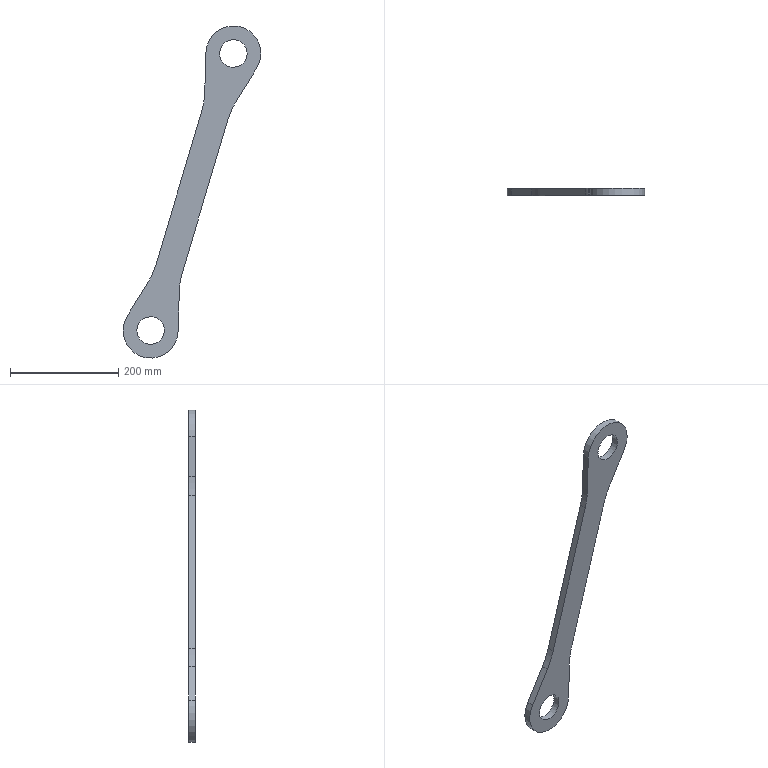Component | NX | CONNECTOR_2_2 | 1 solid | 16 faces | volume 466059 mm3 | plane 8 | cylinder 8 | commonest cylinder face diameters 280 x4 101.6 x2 50.8 x2